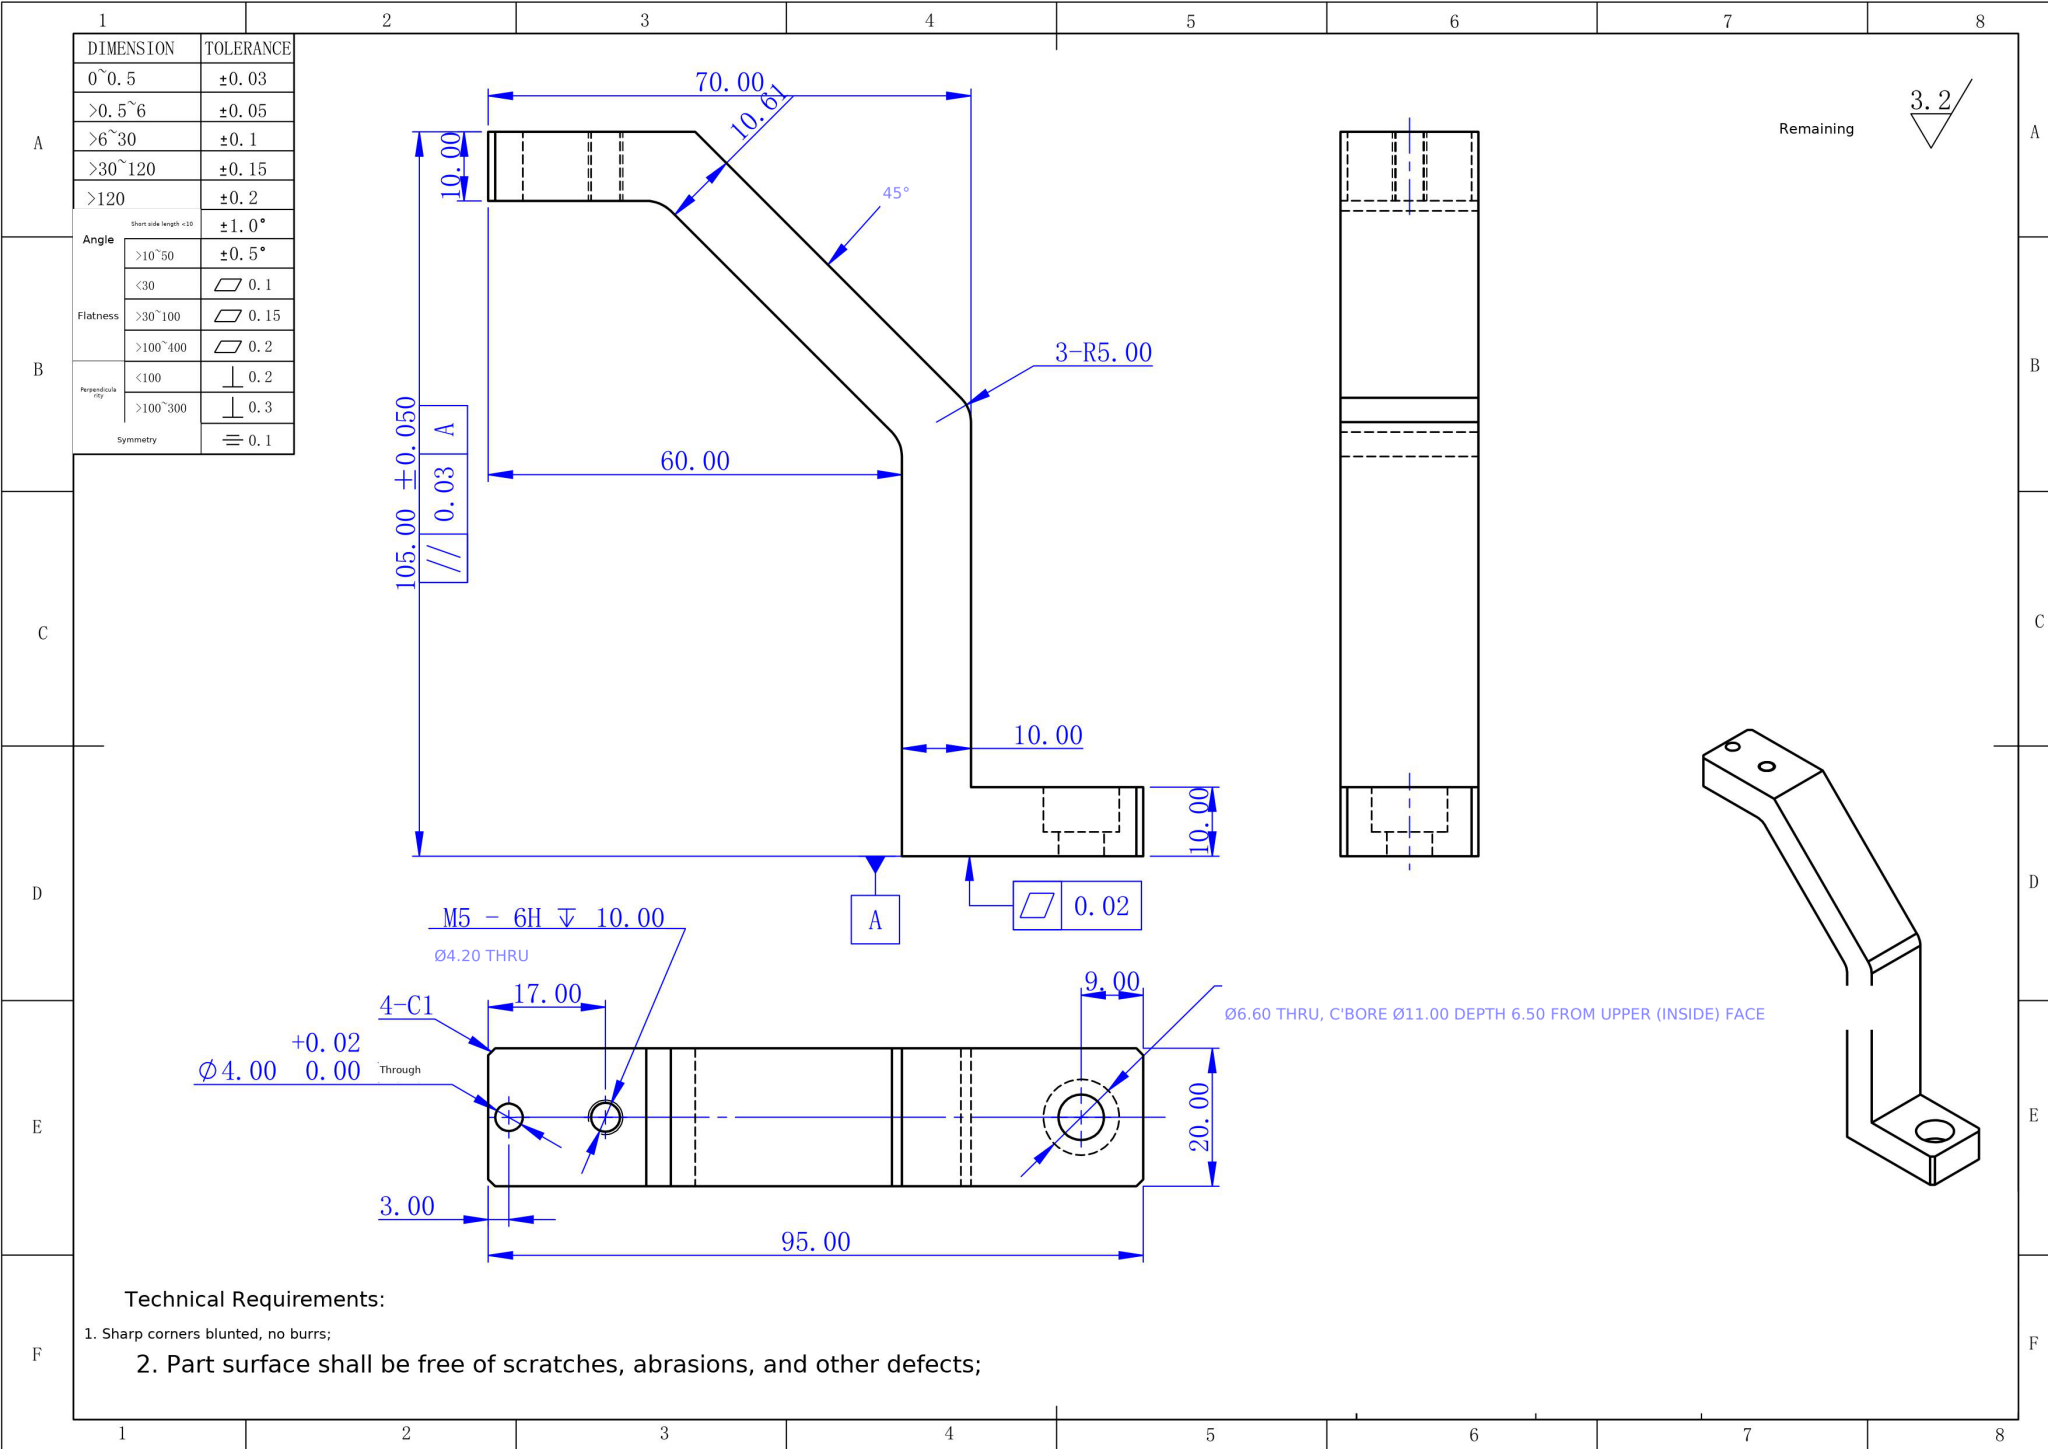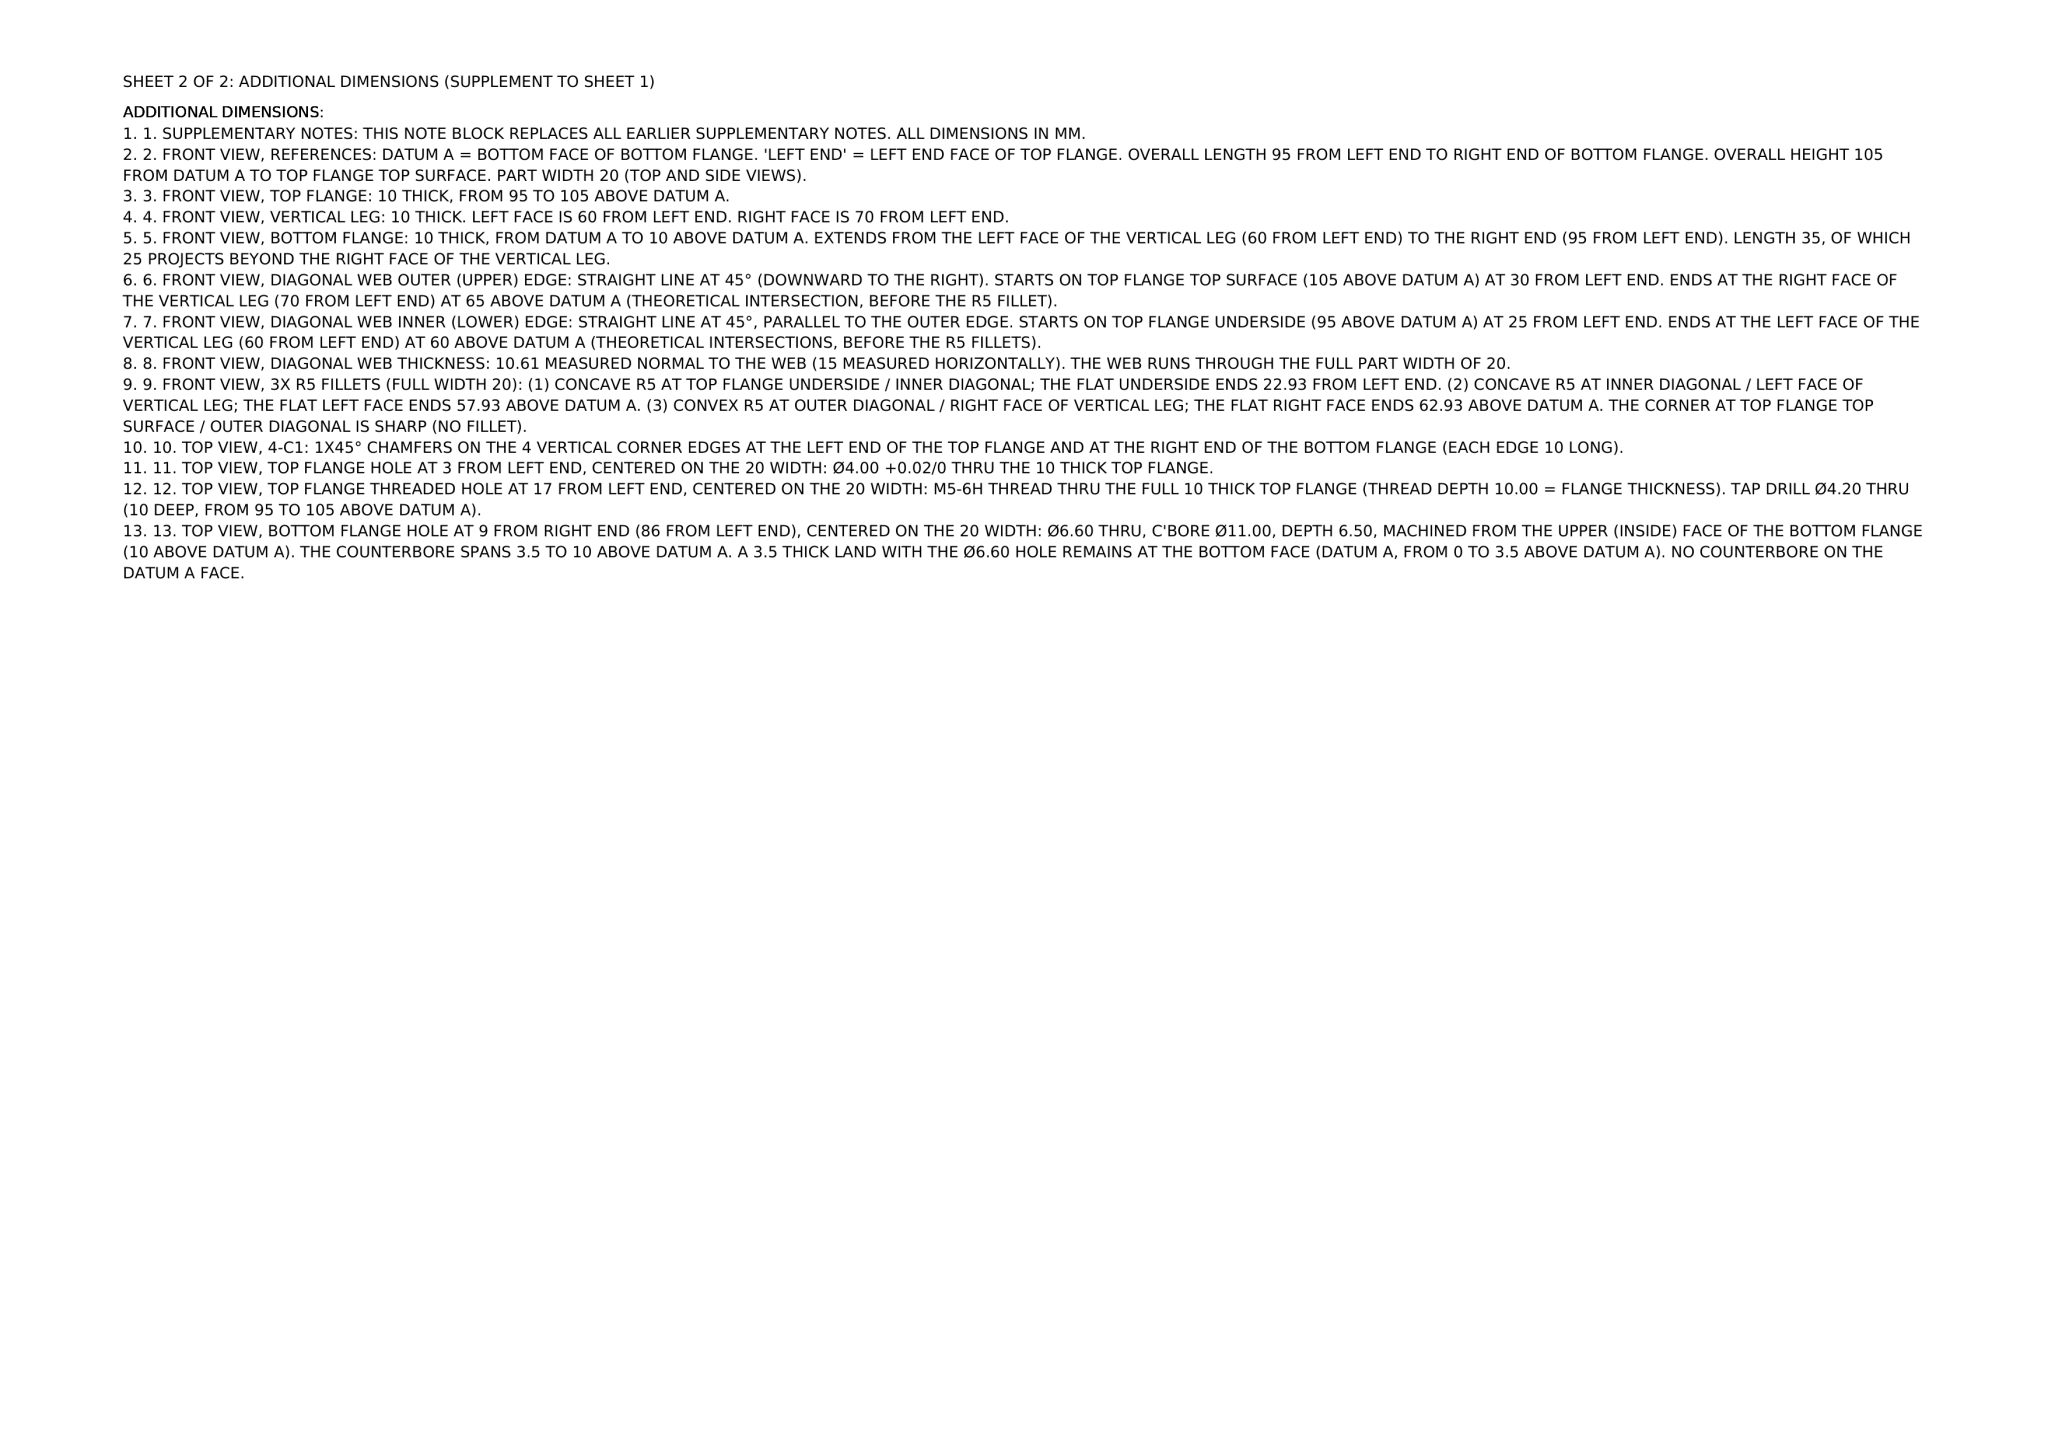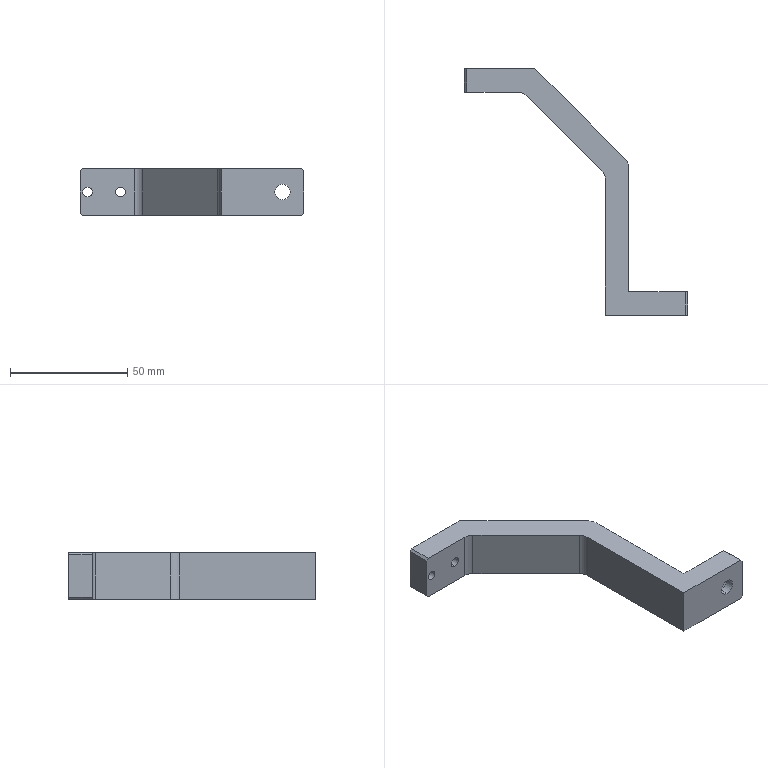Part | NX | mm | 1 solid | 28 faces | box 95 x 105 x 20 mm | volume 33239 mm3 | plane 17 | cylinder 11 | commonest cylinder face diameters 10 x3 4 x2 4.2 x2 11 x2 6.6 x2